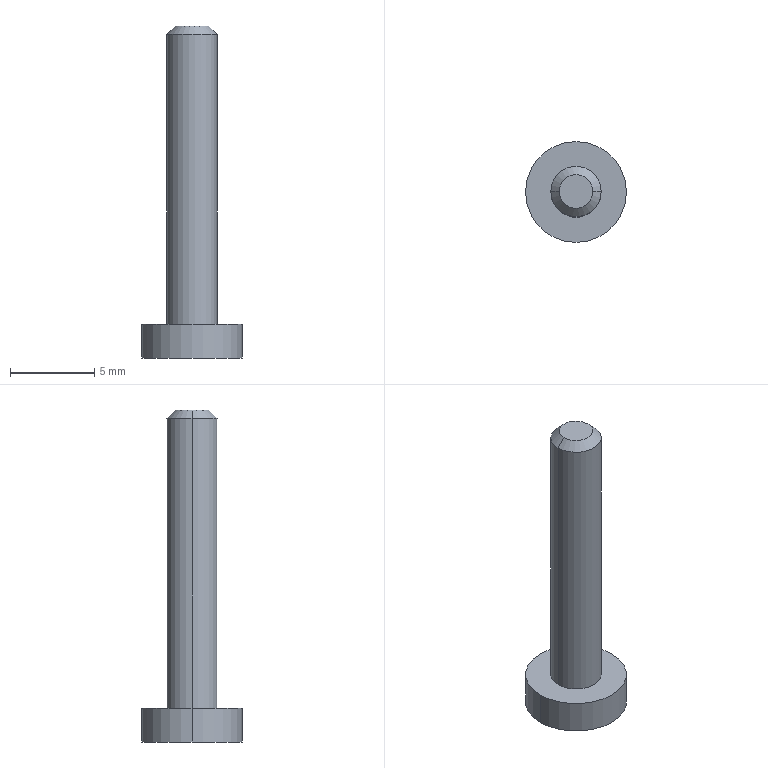Component | SolidWorks | gbgbCJPB6-5-B(0)F8-1_gbgbCJPB6-5-B_RODF8-1 | 1 solid | 9 faces | box 6 x 6 x 19.75 mm | volume 181 mm3 | cylinder 4 | plane 3 | cone 2 | commonest cylinder face diameters 6 x2 3 x2
build123d program:
from build123d import *


with BuildPart() as part:
    # Sketch1 → Revolve1 (revolve)
    with BuildSketch(Plane.XY, mode=Mode.PRIVATE) as revolve1_sk:
        Polygon((-9, 0), (-9, 1), (-8.5, 1.5), (8.75, 1.5), (8.75, 3), (10.75, 3), (10.75, 0), align=None)
    revolve(revolve1_sk.sketch.rotate(Axis((10.75, 0, 0), (-1, 0, 0)), 270), axis=Axis((10.75, 0, 0), (-1, 0, 0)))


solid = part.part

# Placed as in the assembly
solid = solid.moved(Location((61.196, 359.97, 412.732), (0, 90, 0)))
STEP:
#1=COLOUR_RGB('',0.7922,0.8196,0.9333);
#2=FILL_AREA_STYLE_COLOUR('',#1);
#3=FILL_AREA_STYLE('',(#2));
#4=SURFACE_STYLE_FILL_AREA(#3);
#5=SURFACE_SIDE_STYLE('',(#4));
#6=SURFACE_STYLE_USAGE(.BOTH.,#5);
#7=PRESENTATION_STYLE_ASSIGNMENT((#6));
#8=CARTESIAN_POINT('',(2.527,14.172,15.826));
#9=VERTEX_POINT('',#8);
#10=CARTESIAN_POINT('',(2.291,14.172,15.826));
#11=VERTEX_POINT('',#10);
#12=CARTESIAN_POINT('',(2.409,14.172,15.826));
#13=DIRECTION('',(0.,0.,1.));
#14=DIRECTION('',(1.,0.,0.));
#15=AXIS2_PLACEMENT_3D('',#12,#13,#14);
#16=CIRCLE('',#15,0.1181);
#17=EDGE_CURVE('',#9,#11,#16,.T.);
#18=ORIENTED_EDGE('',*,*,#17,.T.);
#19=CARTESIAN_POINT('',(2.291,14.172,15.905));
#20=VERTEX_POINT('',#19);
#21=CARTESIAN_POINT('',(2.291,14.172,15.826));
#22=DIRECTION('',(0.,0.,1.));
#23=VECTOR('',#22,39.37);
#24=LINE('',#21,#23);
#25=EDGE_CURVE('',#11,#20,#24,.T.);
#26=ORIENTED_EDGE('',*,*,#25,.T.);
#27=CARTESIAN_POINT('',(2.527,14.172,15.905));
#28=VERTEX_POINT('',#27);
#29=CARTESIAN_POINT('',(2.409,14.172,15.905));
#30=DIRECTION('',(0.,0.,1.));
#31=DIRECTION('',(1.,0.,0.));
#32=AXIS2_PLACEMENT_3D('',#29,#30,#31);
#33=CIRCLE('',#32,0.1181);
#34=EDGE_CURVE('',#28,#20,#33,.T.);
#35=ORIENTED_EDGE('',*,*,#34,.F.);
#36=CARTESIAN_POINT('',(2.527,14.172,15.826));
#37=DIRECTION('',(0.,0.,1.));
#38=VECTOR('',#37,39.37);
#39=LINE('',#36,#38);
#40=EDGE_CURVE('',#9,#28,#39,.T.);
#41=ORIENTED_EDGE('',*,*,#40,.F.);
#42=EDGE_LOOP('',(#18,#26,#35,#41));
#43=FACE_OUTER_BOUND('',#42,.T.);
#44=CARTESIAN_POINT('',(2.409,14.172,15.826));
#45=DIRECTION('',(0.,0.,1.));
#46=DIRECTION('',(1.,0.,0.));
#47=AXIS2_PLACEMENT_3D('',#44,#45,#46);
#48=CYLINDRICAL_SURFACE('',#47,0.1181);
#49=ADVANCED_FACE('',(#43),#48,.T.);
#50=CARTESIAN_POINT('',(2.468,14.172,15.905));
#51=VERTEX_POINT('',#50);
#52=CARTESIAN_POINT('',(2.35,14.172,15.905));
#53=VERTEX_POINT('',#52);
#54=CARTESIAN_POINT('',(2.409,14.172,15.905));
#55=DIRECTION('',(0.,0.,1.));
#56=DIRECTION('',(1.,0.,0.));
#57=AXIS2_PLACEMENT_3D('',#54,#55,#56);
#58=CIRCLE('',#57,0.05906);
#59=EDGE_CURVE('',#51,#53,#58,.T.);
#60=ORIENTED_EDGE('',*,*,#59,.T.);
#61=CARTESIAN_POINT('',(2.35,14.172,16.584));
#62=VERTEX_POINT('',#61);
#63=CARTESIAN_POINT('',(2.35,14.172,15.826));
#64=DIRECTION('',(0.,0.,1.));
#65=VECTOR('',#64,39.37);
#66=LINE('',#63,#65);
#67=EDGE_CURVE('',#53,#62,#66,.T.);
#68=ORIENTED_EDGE('',*,*,#67,.T.);
#69=CARTESIAN_POINT('',(2.468,14.172,16.584));
#70=VERTEX_POINT('',#69);
#71=CARTESIAN_POINT('',(2.409,14.172,16.584));
#72=DIRECTION('',(0.,0.,1.));
#73=DIRECTION('',(1.,0.,0.));
#74=AXIS2_PLACEMENT_3D('',#71,#72,#73);
#75=CIRCLE('',#74,0.05906);
#76=EDGE_CURVE('',#70,#62,#75,.T.);
#77=ORIENTED_EDGE('',*,*,#76,.F.);
#78=CARTESIAN_POINT('',(2.468,14.172,15.826));
#79=DIRECTION('',(0.,0.,1.));
#80=VECTOR('',#79,39.37);
#81=LINE('',#78,#80);
#82=EDGE_CURVE('',#51,#70,#81,.T.);
#83=ORIENTED_EDGE('',*,*,#82,.F.);
#84=EDGE_LOOP('',(#60,#68,#77,#83));
#85=FACE_OUTER_BOUND('',#84,.T.);
#86=CARTESIAN_POINT('',(2.409,14.172,15.826));
#87=DIRECTION('',(0.,0.,1.));
#88=DIRECTION('',(1.,0.,0.));
#89=AXIS2_PLACEMENT_3D('',#86,#87,#88);
#90=CYLINDRICAL_SURFACE('',#89,0.05906);
#91=ADVANCED_FACE('',(#85),#90,.T.);
#92=CARTESIAN_POINT('',(2.449,14.172,16.604));
#93=VERTEX_POINT('',#92);
#94=CARTESIAN_POINT('',(2.37,14.172,16.604));
#95=VERTEX_POINT('',#94);
#96=CARTESIAN_POINT('',(2.409,14.172,16.604));
#97=DIRECTION('',(0.,0.,1.));
#98=DIRECTION('',(1.,0.,0.));
#99=AXIS2_PLACEMENT_3D('',#96,#97,#98);
#100=CIRCLE('',#99,0.03937);
#101=EDGE_CURVE('',#93,#95,#100,.T.);
#102=ORIENTED_EDGE('',*,*,#101,.F.);
#103=CARTESIAN_POINT('',(2.468,14.172,16.584));
#104=DIRECTION('',(0.7071,-0.,-0.7071));
#105=VECTOR('',#104,39.37);
#106=LINE('',#103,#105);
#107=EDGE_CURVE('',#93,#70,#106,.T.);
#108=ORIENTED_EDGE('',*,*,#107,.T.);
#109=ORIENTED_EDGE('',*,*,#76,.T.);
#110=CARTESIAN_POINT('',(2.35,14.172,16.584));
#111=DIRECTION('',(-0.7071,-0.,-0.7071));
#112=VECTOR('',#111,39.37);
#113=LINE('',#110,#112);
#114=EDGE_CURVE('',#95,#62,#113,.T.);
#115=ORIENTED_EDGE('',*,*,#114,.F.);
#116=EDGE_LOOP('',(#102,#108,#109,#115));
#117=FACE_OUTER_BOUND('',#116,.T.);
#118=CARTESIAN_POINT('',(2.409,14.172,16.584));
#119=DIRECTION('',(0.,-0.,-1.));
#120=DIRECTION('',(-1.,0.,0.));
#121=AXIS2_PLACEMENT_3D('',#118,#119,#120);
#122=CONICAL_SURFACE('',#121,0.05906,0.7854);
#123=ADVANCED_FACE('',(#117),#122,.T.);
#124=CARTESIAN_POINT('',(2.409,14.172,16.604));
#125=DIRECTION('',(0.,0.,1.));
#126=DIRECTION('',(1.,0.,0.));
#127=AXIS2_PLACEMENT_3D('',#124,#125,#126);
#128=CIRCLE('',#127,0.03937);
#129=EDGE_CURVE('',#95,#93,#128,.T.);
#130=ORIENTED_EDGE('',*,*,#129,.T.);
#131=ORIENTED_EDGE('',*,*,#101,.T.);
#132=EDGE_LOOP('',(#130,#131));
#133=FACE_OUTER_BOUND('',#132,.T.);
#134=CARTESIAN_POINT('',(2.409,14.172,16.604));
#135=DIRECTION('',(0.,-0.,-1.));
#136=DIRECTION('',(-1.,0.,-0.));
#137=AXIS2_PLACEMENT_3D('',#134,#135,#136);
#138=PLANE('',#137);
#139=ADVANCED_FACE('',(#133),#138,.F.);
#140=ORIENTED_EDGE('',*,*,#107,.F.);
#141=ORIENTED_EDGE('',*,*,#129,.F.);
#142=ORIENTED_EDGE('',*,*,#114,.T.);
#143=CARTESIAN_POINT('',(2.409,14.172,16.584));
#144=DIRECTION('',(0.,0.,1.));
#145=DIRECTION('',(1.,0.,0.));
#146=AXIS2_PLACEMENT_3D('',#143,#144,#145);
#147=CIRCLE('',#146,0.05906);
#148=EDGE_CURVE('',#62,#70,#147,.T.);
#149=ORIENTED_EDGE('',*,*,#148,.T.);
#150=EDGE_LOOP('',(#140,#141,#142,#149));
#151=FACE_OUTER_BOUND('',#150,.T.);
#152=CARTESIAN_POINT('',(2.409,14.172,16.584));
#153=DIRECTION('',(0.,-0.,-1.));
#154=DIRECTION('',(-1.,0.,0.));
#155=AXIS2_PLACEMENT_3D('',#152,#153,#154);
#156=CONICAL_SURFACE('',#155,0.05906,0.7854);
#157=ADVANCED_FACE('',(#151),#156,.T.);
#158=ORIENTED_EDGE('',*,*,#67,.F.);
#159=CARTESIAN_POINT('',(2.409,14.172,15.905));
#160=DIRECTION('',(0.,0.,1.));
#161=DIRECTION('',(1.,0.,0.));
#162=AXIS2_PLACEMENT_3D('',#159,#160,#161);
#163=CIRCLE('',#162,0.05906);
#164=EDGE_CURVE('',#53,#51,#163,.T.);
#165=ORIENTED_EDGE('',*,*,#164,.T.);
#166=ORIENTED_EDGE('',*,*,#82,.T.);
#167=ORIENTED_EDGE('',*,*,#148,.F.);
#168=EDGE_LOOP('',(#158,#165,#166,#167));
#169=FACE_OUTER_BOUND('',#168,.T.);
#170=CARTESIAN_POINT('',(2.409,14.172,15.826));
#171=DIRECTION('',(0.,0.,1.));
#172=DIRECTION('',(1.,0.,0.));
#173=AXIS2_PLACEMENT_3D('',#170,#171,#172);
#174=CYLINDRICAL_SURFACE('',#173,0.05906);
#175=ADVANCED_FACE('',(#169),#174,.T.);
#176=ORIENTED_EDGE('',*,*,#59,.F.);
#177=ORIENTED_EDGE('',*,*,#164,.F.);
#178=EDGE_LOOP('',(#176,#177));
#179=FACE_BOUND('',#178,.T.);
#180=ORIENTED_EDGE('',*,*,#34,.T.);
#181=CARTESIAN_POINT('',(2.409,14.172,15.905));
#182=DIRECTION('',(0.,0.,1.));
#183=DIRECTION('',(1.,0.,0.));
#184=AXIS2_PLACEMENT_3D('',#181,#182,#183);
#185=CIRCLE('',#184,0.1181);
#186=EDGE_CURVE('',#20,#28,#185,.T.);
#187=ORIENTED_EDGE('',*,*,#186,.T.);
#188=EDGE_LOOP('',(#180,#187));
#189=FACE_OUTER_BOUND('',#188,.T.);
#190=CARTESIAN_POINT('',(2.409,14.231,15.905));
#191=DIRECTION('',(0.,-0.,-1.));
#192=DIRECTION('',(-1.,0.,-0.));
#193=AXIS2_PLACEMENT_3D('',#190,#191,#192);
#194=PLANE('',#193);
#195=ADVANCED_FACE('',(#179,#189),#194,.F.);
#196=ORIENTED_EDGE('',*,*,#25,.F.);
#197=CARTESIAN_POINT('',(2.409,14.172,15.826));
#198=DIRECTION('',(0.,0.,1.));
#199=DIRECTION('',(1.,0.,0.));
#200=AXIS2_PLACEMENT_3D('',#197,#198,#199);
#201=CIRCLE('',#200,0.1181);
#202=EDGE_CURVE('',#11,#9,#201,.T.);
#203=ORIENTED_EDGE('',*,*,#202,.T.);
#204=ORIENTED_EDGE('',*,*,#40,.T.);
#205=ORIENTED_EDGE('',*,*,#186,.F.);
#206=EDGE_LOOP('',(#196,#203,#204,#205));
#207=FACE_OUTER_BOUND('',#206,.T.);
#208=CARTESIAN_POINT('',(2.409,14.172,15.826));
#209=DIRECTION('',(0.,0.,1.));
#210=DIRECTION('',(1.,0.,0.));
#211=AXIS2_PLACEMENT_3D('',#208,#209,#210);
#212=CYLINDRICAL_SURFACE('',#211,0.1181);
#213=ADVANCED_FACE('',(#207),#212,.T.);
#214=ORIENTED_EDGE('',*,*,#17,.F.);
#215=ORIENTED_EDGE('',*,*,#202,.F.);
#216=EDGE_LOOP('',(#214,#215));
#217=FACE_OUTER_BOUND('',#216,.T.);
#218=CARTESIAN_POINT('',(2.409,14.29,15.826));
#219=DIRECTION('',(0.,0.,1.));
#220=DIRECTION('',(1.,-0.,0.));
#221=AXIS2_PLACEMENT_3D('',#218,#219,#220);
#222=PLANE('',#221);
#223=ADVANCED_FACE('',(#217),#222,.F.);
#224=CLOSED_SHELL('',(#49,#91,#123,#139,#157,#175,#195,#213,#223));
#225=MANIFOLD_SOLID_BREP('',#224);
#226=STYLED_ITEM('',(#7),#225);
#227=(LENGTH_UNIT()NAMED_UNIT(*)SI_UNIT($,.METRE.));
#228=LENGTH_MEASURE_WITH_UNIT(LENGTH_MEASURE(0.0254),#227);
#229=DIMENSIONAL_EXPONENTS(1.,0.,0.,0.,0.,0.,0.);
#230=(CONVERSION_BASED_UNIT('',#228)LENGTH_UNIT()NAMED_UNIT(#229));
#231=UNCERTAINTY_MEASURE_WITH_UNIT(LENGTH_MEASURE(0.00001),#230,'','');
#232=(NAMED_UNIT(*)PLANE_ANGLE_UNIT()SI_UNIT($,.RADIAN.));
#233=(NAMED_UNIT(*)SI_UNIT($,.STERADIAN.)SOLID_ANGLE_UNIT());
#234=(GEOMETRIC_REPRESENTATION_CONTEXT(3)GLOBAL_UNCERTAINTY_ASSIGNED_CONTEXT((#231))GLOBAL_UNIT_ASSIGNED_CONTEXT((#230,#232,#233))REPRESENTATION_CONTEXT('',''));
#235=MECHANICAL_DESIGN_GEOMETRIC_PRESENTATION_REPRESENTATION('',(#226),#234);
#236=CARTESIAN_POINT('',(0.,0.,0.));
#237=DIRECTION('',(0.,0.,1.));
#238=DIRECTION('',(1.,0.,0.));
#239=AXIS2_PLACEMENT_3D('',#236,#237,#238);
#240=(LENGTH_UNIT()NAMED_UNIT(*)SI_UNIT($,.METRE.));
#241=LENGTH_MEASURE_WITH_UNIT(LENGTH_MEASURE(0.0254),#240);
#242=DIMENSIONAL_EXPONENTS(1.,0.,0.,0.,0.,0.,0.);
#243=(CONVERSION_BASED_UNIT('',#241)LENGTH_UNIT()NAMED_UNIT(#242));
#244=UNCERTAINTY_MEASURE_WITH_UNIT(LENGTH_MEASURE(0.00001),#243,'','');
#245=(NAMED_UNIT(*)PLANE_ANGLE_UNIT()SI_UNIT($,.RADIAN.));
#246=(NAMED_UNIT(*)SI_UNIT($,.STERADIAN.)SOLID_ANGLE_UNIT());
#247=(GEOMETRIC_REPRESENTATION_CONTEXT(3)GLOBAL_UNCERTAINTY_ASSIGNED_CONTEXT((#244))GLOBAL_UNIT_ASSIGNED_CONTEXT((#243,#245,#246))REPRESENTATION_CONTEXT('',''));
#248=ADVANCED_BREP_SHAPE_REPRESENTATION('',(#225,#239),#247);
#249=PRESENTATION_LAYER_ASSIGNMENT('','',(#226));